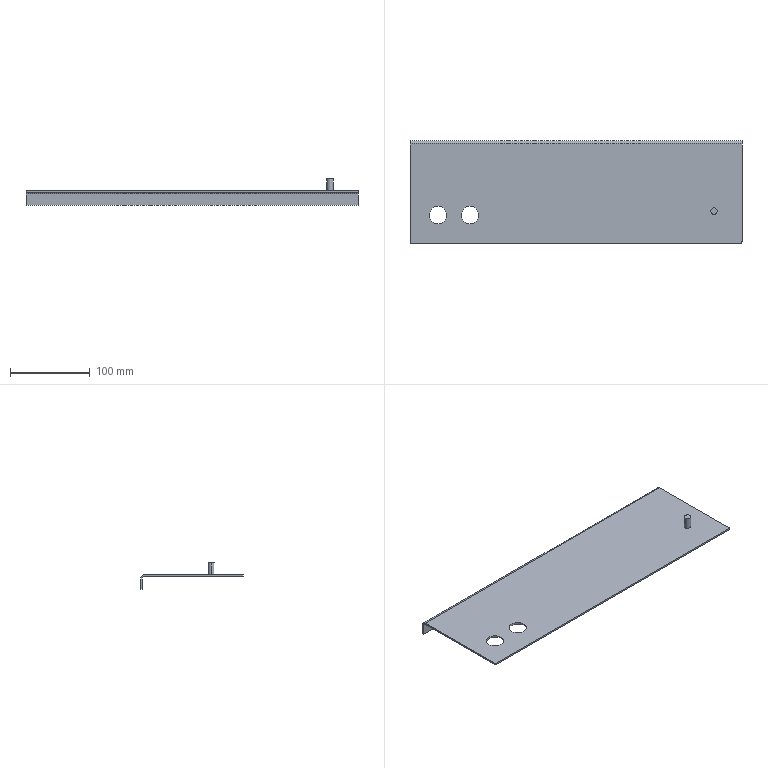Component | SolidWorks | ElectricalCabinetAssembly-1_CabinetAssembly-1_ElectricalCabinetBaffle-1 | 1 solid | 23 faces | box 415 x 128 x 33 mm | volume 117681 mm3 | plane 13 | cylinder 10 | commonest cylinder face diameters 22 x4 8 x3 4 x3 | material Plain Carbon Steel
STEP:
#1=COLOUR_RGB('',0.7922,0.8196,0.9333);
#2=FILL_AREA_STYLE_COLOUR('',#1);
#3=FILL_AREA_STYLE('',(#2));
#4=SURFACE_STYLE_FILL_AREA(#3);
#5=SURFACE_SIDE_STYLE('',(#4));
#6=SURFACE_STYLE_USAGE(.BOTH.,#5);
#7=PRESENTATION_STYLE_ASSIGNMENT((#6));
#8=CARTESIAN_POINT('',(94.303,43.919,55.885));
#9=VERTEX_POINT('',#8);
#10=CARTESIAN_POINT('',(93.988,43.919,55.885));
#11=VERTEX_POINT('',#10);
#12=CARTESIAN_POINT('',(94.145,43.919,55.885));
#13=DIRECTION('',(0.,-0.,1.));
#14=DIRECTION('',(1.,0.,0.));
#15=AXIS2_PLACEMENT_3D('',#12,#13,#14);
#16=CIRCLE('',#15,0.1575);
#17=EDGE_CURVE('',#9,#11,#16,.T.);
#18=ORIENTED_EDGE('',*,*,#17,.F.);
#19=CARTESIAN_POINT('',(94.303,43.919,55.294));
#20=VERTEX_POINT('',#19);
#21=CARTESIAN_POINT('',(94.303,43.919,55.885));
#22=DIRECTION('',(-0.,0.,-1.));
#23=VECTOR('',#22,39.37);
#24=LINE('',#21,#23);
#25=EDGE_CURVE('',#9,#20,#24,.T.);
#26=ORIENTED_EDGE('',*,*,#25,.T.);
#27=CARTESIAN_POINT('',(93.988,43.919,55.294));
#28=VERTEX_POINT('',#27);
#29=CARTESIAN_POINT('',(94.145,43.919,55.294));
#30=DIRECTION('',(0.,-0.,1.));
#31=DIRECTION('',(1.,0.,0.));
#32=AXIS2_PLACEMENT_3D('',#29,#30,#31);
#33=CIRCLE('',#32,0.1575);
#34=EDGE_CURVE('',#20,#28,#33,.T.);
#35=ORIENTED_EDGE('',*,*,#34,.T.);
#36=CARTESIAN_POINT('',(93.988,43.919,55.885));
#37=DIRECTION('',(-0.,0.,-1.));
#38=VECTOR('',#37,39.37);
#39=LINE('',#36,#38);
#40=EDGE_CURVE('',#11,#28,#39,.T.);
#41=ORIENTED_EDGE('',*,*,#40,.F.);
#42=EDGE_LOOP('',(#18,#26,#35,#41));
#43=FACE_OUTER_BOUND('',#42,.T.);
#44=CARTESIAN_POINT('',(94.145,43.919,55.885));
#45=DIRECTION('',(-0.,0.,-1.));
#46=DIRECTION('',(-1.,0.,0.));
#47=AXIS2_PLACEMENT_3D('',#44,#45,#46);
#48=CYLINDRICAL_SURFACE('',#47,0.1575);
#49=ADVANCED_FACE('',(#43),#48,.T.);
#50=CARTESIAN_POINT('',(81.704,43.722,55.216));
#51=VERTEX_POINT('',#50);
#52=CARTESIAN_POINT('',(82.57,43.722,55.216));
#53=VERTEX_POINT('',#52);
#54=CARTESIAN_POINT('',(82.137,43.722,55.216));
#55=DIRECTION('',(0.,-0.,1.));
#56=DIRECTION('',(1.,0.,0.));
#57=AXIS2_PLACEMENT_3D('',#54,#55,#56);
#58=CIRCLE('',#57,0.4331);
#59=EDGE_CURVE('',#51,#53,#58,.T.);
#60=ORIENTED_EDGE('',*,*,#59,.F.);
#61=CARTESIAN_POINT('',(81.704,43.722,55.294));
#62=VERTEX_POINT('',#61);
#63=CARTESIAN_POINT('',(81.704,43.722,54.901));
#64=DIRECTION('',(0.,-0.,1.));
#65=VECTOR('',#64,39.37);
#66=LINE('',#63,#65);
#67=EDGE_CURVE('',#51,#62,#66,.T.);
#68=ORIENTED_EDGE('',*,*,#67,.T.);
#69=CARTESIAN_POINT('',(82.57,43.722,55.294));
#70=VERTEX_POINT('',#69);
#71=CARTESIAN_POINT('',(82.137,43.722,55.294));
#72=DIRECTION('',(0.,-0.,1.));
#73=DIRECTION('',(1.,0.,0.));
#74=AXIS2_PLACEMENT_3D('',#71,#72,#73);
#75=CIRCLE('',#74,0.4331);
#76=EDGE_CURVE('',#62,#70,#75,.T.);
#77=ORIENTED_EDGE('',*,*,#76,.T.);
#78=CARTESIAN_POINT('',(82.57,43.722,54.901));
#79=DIRECTION('',(0.,-0.,1.));
#80=VECTOR('',#79,39.37);
#81=LINE('',#78,#80);
#82=EDGE_CURVE('',#53,#70,#81,.T.);
#83=ORIENTED_EDGE('',*,*,#82,.F.);
#84=EDGE_LOOP('',(#60,#68,#77,#83));
#85=FACE_OUTER_BOUND('',#84,.T.);
#86=CARTESIAN_POINT('',(82.137,43.722,54.901));
#87=DIRECTION('',(0.,-0.,1.));
#88=DIRECTION('',(1.,0.,0.));
#89=AXIS2_PLACEMENT_3D('',#86,#87,#88);
#90=CYLINDRICAL_SURFACE('',#89,0.4331);
#91=ADVANCED_FACE('',(#85),#90,.F.);
#92=CARTESIAN_POINT('',(80.129,43.722,55.216));
#93=VERTEX_POINT('',#92);
#94=CARTESIAN_POINT('',(80.996,43.722,55.216));
#95=VERTEX_POINT('',#94);
#96=CARTESIAN_POINT('',(80.562,43.722,55.216));
#97=DIRECTION('',(0.,-0.,1.));
#98=DIRECTION('',(1.,0.,0.));
#99=AXIS2_PLACEMENT_3D('',#96,#97,#98);
#100=CIRCLE('',#99,0.4331);
#101=EDGE_CURVE('',#93,#95,#100,.T.);
#102=ORIENTED_EDGE('',*,*,#101,.F.);
#103=CARTESIAN_POINT('',(80.129,43.722,55.294));
#104=VERTEX_POINT('',#103);
#105=CARTESIAN_POINT('',(80.129,43.722,54.901));
#106=DIRECTION('',(0.,-0.,1.));
#107=VECTOR('',#106,39.37);
#108=LINE('',#105,#107);
#109=EDGE_CURVE('',#93,#104,#108,.T.);
#110=ORIENTED_EDGE('',*,*,#109,.T.);
#111=CARTESIAN_POINT('',(80.996,43.722,55.294));
#112=VERTEX_POINT('',#111);
#113=CARTESIAN_POINT('',(80.562,43.722,55.294));
#114=DIRECTION('',(0.,-0.,1.));
#115=DIRECTION('',(1.,0.,0.));
#116=AXIS2_PLACEMENT_3D('',#113,#114,#115);
#117=CIRCLE('',#116,0.4331);
#118=EDGE_CURVE('',#104,#112,#117,.T.);
#119=ORIENTED_EDGE('',*,*,#118,.T.);
#120=CARTESIAN_POINT('',(80.996,43.722,54.901));
#121=DIRECTION('',(0.,-0.,1.));
#122=VECTOR('',#121,39.37);
#123=LINE('',#120,#122);
#124=EDGE_CURVE('',#95,#112,#123,.T.);
#125=ORIENTED_EDGE('',*,*,#124,.F.);
#126=EDGE_LOOP('',(#102,#110,#119,#125));
#127=FACE_OUTER_BOUND('',#126,.T.);
#128=CARTESIAN_POINT('',(80.562,43.722,54.901));
#129=DIRECTION('',(0.,-0.,1.));
#130=DIRECTION('',(1.,0.,0.));
#131=AXIS2_PLACEMENT_3D('',#128,#129,#130);
#132=CYLINDRICAL_SURFACE('',#131,0.4331);
#133=ADVANCED_FACE('',(#127),#132,.F.);
#134=CARTESIAN_POINT('',(95.523,47.226,55.216));
#135=VERTEX_POINT('',#134);
#136=CARTESIAN_POINT('',(95.523,42.423,55.216));
#137=VERTEX_POINT('',#136);
#138=CARTESIAN_POINT('',(95.523,42.423,55.216));
#139=DIRECTION('',(0.,-1.,-0.));
#140=VECTOR('',#139,39.37);
#141=LINE('',#138,#140);
#142=EDGE_CURVE('',#135,#137,#141,.T.);
#143=ORIENTED_EDGE('',*,*,#142,.F.);
#144=CARTESIAN_POINT('',(95.523,47.226,55.294));
#145=VERTEX_POINT('',#144);
#146=CARTESIAN_POINT('',(95.523,47.226,55.216));
#147=DIRECTION('',(0.,-0.,1.));
#148=VECTOR('',#147,39.37);
#149=LINE('',#146,#148);
#150=EDGE_CURVE('',#135,#145,#149,.T.);
#151=ORIENTED_EDGE('',*,*,#150,.T.);
#152=CARTESIAN_POINT('',(95.523,42.423,55.294));
#153=VERTEX_POINT('',#152);
#154=CARTESIAN_POINT('',(95.523,42.423,55.294));
#155=DIRECTION('',(0.,-1.,-0.));
#156=VECTOR('',#155,39.37);
#157=LINE('',#154,#156);
#158=EDGE_CURVE('',#145,#153,#157,.T.);
#159=ORIENTED_EDGE('',*,*,#158,.T.);
#160=CARTESIAN_POINT('',(95.523,42.423,55.294));
#161=DIRECTION('',(-0.,0.,-1.));
#162=VECTOR('',#161,39.37);
#163=LINE('',#160,#162);
#164=EDGE_CURVE('',#153,#137,#163,.T.);
#165=ORIENTED_EDGE('',*,*,#164,.T.);
#166=EDGE_LOOP('',(#143,#151,#159,#165));
#167=FACE_OUTER_BOUND('',#166,.T.);
#168=CARTESIAN_POINT('',(95.523,42.423,55.294));
#169=DIRECTION('',(1.,0.,-0.));
#170=DIRECTION('',(-0.,0.,-1.));
#171=AXIS2_PLACEMENT_3D('',#168,#169,#170);
#172=PLANE('',#171);
#173=ADVANCED_FACE('',(#167),#172,.T.);
#174=CARTESIAN_POINT('',(94.145,43.919,55.294));
#175=DIRECTION('',(0.,-0.,1.));
#176=DIRECTION('',(1.,0.,0.));
#177=AXIS2_PLACEMENT_3D('',#174,#175,#176);
#178=CIRCLE('',#177,0.1575);
#179=EDGE_CURVE('',#28,#20,#178,.T.);
#180=ORIENTED_EDGE('',*,*,#179,.F.);
#181=ORIENTED_EDGE('',*,*,#34,.F.);
#182=EDGE_LOOP('',(#180,#181));
#183=FACE_BOUND('',#182,.T.);
#184=CARTESIAN_POINT('',(82.137,43.722,55.294));
#185=DIRECTION('',(0.,-0.,1.));
#186=DIRECTION('',(1.,0.,0.));
#187=AXIS2_PLACEMENT_3D('',#184,#185,#186);
#188=CIRCLE('',#187,0.4331);
#189=EDGE_CURVE('',#70,#62,#188,.T.);
#190=ORIENTED_EDGE('',*,*,#189,.F.);
#191=ORIENTED_EDGE('',*,*,#76,.F.);
#192=EDGE_LOOP('',(#190,#191));
#193=FACE_BOUND('',#192,.T.);
#194=CARTESIAN_POINT('',(80.562,43.722,55.294));
#195=DIRECTION('',(0.,-0.,1.));
#196=DIRECTION('',(1.,0.,0.));
#197=AXIS2_PLACEMENT_3D('',#194,#195,#196);
#198=CIRCLE('',#197,0.4331);
#199=EDGE_CURVE('',#112,#104,#198,.T.);
#200=ORIENTED_EDGE('',*,*,#199,.F.);
#201=ORIENTED_EDGE('',*,*,#118,.F.);
#202=EDGE_LOOP('',(#200,#201));
#203=FACE_BOUND('',#202,.T.);
#204=ORIENTED_EDGE('',*,*,#158,.F.);
#205=CARTESIAN_POINT('',(79.185,47.226,55.294));
#206=VERTEX_POINT('',#205);
#207=CARTESIAN_POINT('',(95.523,47.226,55.294));
#208=DIRECTION('',(-1.,-0.,0.));
#209=VECTOR('',#208,39.37);
#210=LINE('',#207,#209);
#211=EDGE_CURVE('',#145,#206,#210,.T.);
#212=ORIENTED_EDGE('',*,*,#211,.T.);
#213=CARTESIAN_POINT('',(79.185,42.423,55.294));
#214=VERTEX_POINT('',#213);
#215=CARTESIAN_POINT('',(79.185,42.423,55.294));
#216=DIRECTION('',(-0.,1.,0.));
#217=VECTOR('',#216,39.37);
#218=LINE('',#215,#217);
#219=EDGE_CURVE('',#214,#206,#218,.T.);
#220=ORIENTED_EDGE('',*,*,#219,.F.);
#221=CARTESIAN_POINT('',(79.263,42.344,55.294));
#222=VERTEX_POINT('',#221);
#223=CARTESIAN_POINT('',(79.263,42.423,55.294));
#224=DIRECTION('',(-0.,0.,-1.));
#225=DIRECTION('',(1.,0.,0.));
#226=AXIS2_PLACEMENT_3D('',#223,#224,#225);
#227=CIRCLE('',#226,0.07874);
#228=EDGE_CURVE('',#222,#214,#227,.T.);
#229=ORIENTED_EDGE('',*,*,#228,.F.);
#230=CARTESIAN_POINT('',(95.444,42.344,55.294));
#231=VERTEX_POINT('',#230);
#232=CARTESIAN_POINT('',(95.444,42.344,55.294));
#233=DIRECTION('',(-1.,-0.,0.));
#234=VECTOR('',#233,39.37);
#235=LINE('',#232,#234);
#236=EDGE_CURVE('',#231,#222,#235,.T.);
#237=ORIENTED_EDGE('',*,*,#236,.F.);
#238=CARTESIAN_POINT('',(95.444,42.423,55.294));
#239=DIRECTION('',(-0.,0.,-1.));
#240=DIRECTION('',(1.,0.,0.));
#241=AXIS2_PLACEMENT_3D('',#238,#239,#240);
#242=CIRCLE('',#241,0.07874);
#243=EDGE_CURVE('',#153,#231,#242,.T.);
#244=ORIENTED_EDGE('',*,*,#243,.F.);
#245=EDGE_LOOP('',(#204,#212,#220,#229,#237,#244));
#246=FACE_OUTER_BOUND('',#245,.T.);
#247=CARTESIAN_POINT('',(95.444,42.423,55.294));
#248=DIRECTION('',(0.,-0.,1.));
#249=DIRECTION('',(1.,0.,-0.));
#250=AXIS2_PLACEMENT_3D('',#247,#248,#249);
#251=PLANE('',#250);
#252=ADVANCED_FACE('',(#183,#193,#203,#246),#251,.T.);
#253=CARTESIAN_POINT('',(82.137,43.722,55.216));
#254=DIRECTION('',(0.,-0.,1.));
#255=DIRECTION('',(1.,0.,0.));
#256=AXIS2_PLACEMENT_3D('',#253,#254,#255);
#257=CIRCLE('',#256,0.4331);
#258=EDGE_CURVE('',#53,#51,#257,.T.);
#259=ORIENTED_EDGE('',*,*,#258,.T.);
#260=ORIENTED_EDGE('',*,*,#59,.T.);
#261=EDGE_LOOP('',(#259,#260));
#262=FACE_BOUND('',#261,.T.);
#263=CARTESIAN_POINT('',(80.562,43.722,55.216));
#264=DIRECTION('',(0.,-0.,1.));
#265=DIRECTION('',(1.,0.,0.));
#266=AXIS2_PLACEMENT_3D('',#263,#264,#265);
#267=CIRCLE('',#266,0.4331);
#268=EDGE_CURVE('',#95,#93,#267,.T.);
#269=ORIENTED_EDGE('',*,*,#268,.T.);
#270=ORIENTED_EDGE('',*,*,#101,.T.);
#271=EDGE_LOOP('',(#269,#270));
#272=FACE_BOUND('',#271,.T.);
#273=CARTESIAN_POINT('',(79.185,47.226,55.216));
#274=VERTEX_POINT('',#273);
#275=CARTESIAN_POINT('',(95.523,47.226,55.216));
#276=DIRECTION('',(-1.,-0.,0.));
#277=VECTOR('',#276,39.37);
#278=LINE('',#275,#277);
#279=EDGE_CURVE('',#135,#274,#278,.T.);
#280=ORIENTED_EDGE('',*,*,#279,.F.);
#281=ORIENTED_EDGE('',*,*,#142,.T.);
#282=CARTESIAN_POINT('',(95.444,42.344,55.216));
#283=VERTEX_POINT('',#282);
#284=CARTESIAN_POINT('',(95.444,42.423,55.216));
#285=DIRECTION('',(-0.,0.,-1.));
#286=DIRECTION('',(1.,0.,0.));
#287=AXIS2_PLACEMENT_3D('',#284,#285,#286);
#288=CIRCLE('',#287,0.07874);
#289=EDGE_CURVE('',#137,#283,#288,.T.);
#290=ORIENTED_EDGE('',*,*,#289,.T.);
#291=CARTESIAN_POINT('',(79.263,42.344,55.216));
#292=VERTEX_POINT('',#291);
#293=CARTESIAN_POINT('',(95.444,42.344,55.216));
#294=DIRECTION('',(-1.,-0.,0.));
#295=VECTOR('',#294,39.37);
#296=LINE('',#293,#295);
#297=EDGE_CURVE('',#283,#292,#296,.T.);
#298=ORIENTED_EDGE('',*,*,#297,.T.);
#299=CARTESIAN_POINT('',(79.185,42.423,55.216));
#300=VERTEX_POINT('',#299);
#301=CARTESIAN_POINT('',(79.263,42.423,55.216));
#302=DIRECTION('',(-0.,0.,-1.));
#303=DIRECTION('',(1.,0.,0.));
#304=AXIS2_PLACEMENT_3D('',#301,#302,#303);
#305=CIRCLE('',#304,0.07874);
#306=EDGE_CURVE('',#292,#300,#305,.T.);
#307=ORIENTED_EDGE('',*,*,#306,.T.);
#308=CARTESIAN_POINT('',(79.185,42.423,55.216));
#309=DIRECTION('',(-0.,1.,0.));
#310=VECTOR('',#309,39.37);
#311=LINE('',#308,#310);
#312=EDGE_CURVE('',#300,#274,#311,.T.);
#313=ORIENTED_EDGE('',*,*,#312,.T.);
#314=EDGE_LOOP('',(#280,#281,#290,#298,#307,#313));
#315=FACE_OUTER_BOUND('',#314,.T.);
#316=CARTESIAN_POINT('',(95.444,42.423,55.216));
#317=DIRECTION('',(0.,-0.,1.));
#318=DIRECTION('',(1.,0.,-0.));
#319=AXIS2_PLACEMENT_3D('',#316,#317,#318);
#320=PLANE('',#319);
#321=ADVANCED_FACE('',(#262,#272,#315),#320,.F.);
#322=CARTESIAN_POINT('',(79.185,47.226,55.216));
#323=DIRECTION('',(0.,-0.,1.));
#324=VECTOR('',#323,39.37);
#325=LINE('',#322,#324);
#326=EDGE_CURVE('',#274,#206,#325,.T.);
#327=ORIENTED_EDGE('',*,*,#326,.F.);
#328=ORIENTED_EDGE('',*,*,#312,.F.);
#329=CARTESIAN_POINT('',(79.185,42.423,55.294));
#330=DIRECTION('',(-0.,0.,-1.));
#331=VECTOR('',#330,39.37);
#332=LINE('',#329,#331);
#333=EDGE_CURVE('',#214,#300,#332,.T.);
#334=ORIENTED_EDGE('',*,*,#333,.F.);
#335=ORIENTED_EDGE('',*,*,#219,.T.);
#336=EDGE_LOOP('',(#327,#328,#334,#335));
#337=FACE_OUTER_BOUND('',#336,.T.);
#338=CARTESIAN_POINT('',(79.185,42.423,55.294));
#339=DIRECTION('',(-1.,-0.,0.));
#340=DIRECTION('',(0.,-0.,1.));
#341=AXIS2_PLACEMENT_3D('',#338,#339,#340);
#342=PLANE('',#341);
#343=ADVANCED_FACE('',(#337),#342,.T.);
#344=ORIENTED_EDGE('',*,*,#306,.F.);
#345=CARTESIAN_POINT('',(79.263,42.344,55.294));
#346=DIRECTION('',(-0.,0.,-1.));
#347=VECTOR('',#346,39.37);
#348=LINE('',#345,#347);
#349=EDGE_CURVE('',#222,#292,#348,.T.);
#350=ORIENTED_EDGE('',*,*,#349,.F.);
#351=ORIENTED_EDGE('',*,*,#228,.T.);
#352=ORIENTED_EDGE('',*,*,#333,.T.);
#353=EDGE_LOOP('',(#344,#350,#351,#352));
#354=FACE_OUTER_BOUND('',#353,.T.);
#355=CARTESIAN_POINT('',(79.263,42.423,55.294));
#356=DIRECTION('',(-0.,0.,-1.));
#357=DIRECTION('',(-1.,0.,0.));
#358=AXIS2_PLACEMENT_3D('',#355,#356,#357);
#359=CYLINDRICAL_SURFACE('',#358,0.07874);
#360=ADVANCED_FACE('',(#354),#359,.T.);
#361=ORIENTED_EDGE('',*,*,#297,.F.);
#362=CARTESIAN_POINT('',(95.444,42.344,55.294));
#363=DIRECTION('',(-0.,0.,-1.));
#364=VECTOR('',#363,39.37);
#365=LINE('',#362,#364);
#366=EDGE_CURVE('',#231,#283,#365,.T.);
#367=ORIENTED_EDGE('',*,*,#366,.F.);
#368=ORIENTED_EDGE('',*,*,#236,.T.);
#369=ORIENTED_EDGE('',*,*,#349,.T.);
#370=EDGE_LOOP('',(#361,#367,#368,#369));
#371=FACE_OUTER_BOUND('',#370,.T.);
#372=CARTESIAN_POINT('',(95.444,42.344,55.294));
#373=DIRECTION('',(0.,-1.,-0.));
#374=DIRECTION('',(0.,-0.,1.));
#375=AXIS2_PLACEMENT_3D('',#372,#373,#374);
#376=PLANE('',#375);
#377=ADVANCED_FACE('',(#371),#376,.T.);
#378=ORIENTED_EDGE('',*,*,#289,.F.);
#379=ORIENTED_EDGE('',*,*,#164,.F.);
#380=ORIENTED_EDGE('',*,*,#243,.T.);
#381=ORIENTED_EDGE('',*,*,#366,.T.);
#382=EDGE_LOOP('',(#378,#379,#380,#381));
#383=FACE_OUTER_BOUND('',#382,.T.);
#384=CARTESIAN_POINT('',(95.444,42.423,55.294));
#385=DIRECTION('',(-0.,0.,-1.));
#386=DIRECTION('',(-1.,0.,0.));
#387=AXIS2_PLACEMENT_3D('',#384,#385,#386);
#388=CYLINDRICAL_SURFACE('',#387,0.07874);
#389=ADVANCED_FACE('',(#383),#388,.T.);
#390=CARTESIAN_POINT('',(79.185,47.305,55.137));
#391=VERTEX_POINT('',#390);
#392=CARTESIAN_POINT('',(79.185,47.384,55.137));
#393=VERTEX_POINT('',#392);
#394=CARTESIAN_POINT('',(79.185,47.384,55.137));
#395=DIRECTION('',(-0.,1.,0.));
#396=VECTOR('',#395,39.37);
#397=LINE('',#394,#396);
#398=EDGE_CURVE('',#391,#393,#397,.T.);
#399=ORIENTED_EDGE('',*,*,#398,.F.);
#400=CARTESIAN_POINT('',(79.185,47.226,55.137));
#401=DIRECTION('',(-1.,-0.,0.));
#402=DIRECTION('',(0.,0.,-1.));
#403=AXIS2_PLACEMENT_3D('',#400,#401,#402);
#404=CIRCLE('',#403,0.07874);
#405=EDGE_CURVE('',#274,#391,#404,.T.);
#406=ORIENTED_EDGE('',*,*,#405,.F.);
#407=ORIENTED_EDGE('',*,*,#326,.T.);
#408=CARTESIAN_POINT('',(79.185,47.226,55.137));
#409=DIRECTION('',(-1.,-0.,0.));
#410=DIRECTION('',(0.,0.,-1.));
#411=AXIS2_PLACEMENT_3D('',#408,#409,#410);
#412=CIRCLE('',#411,0.1575);
#413=EDGE_CURVE('',#206,#393,#412,.T.);
#414=ORIENTED_EDGE('',*,*,#413,.T.);
#415=EDGE_LOOP('',(#399,#406,#407,#414));
#416=FACE_OUTER_BOUND('',#415,.T.);
#417=CARTESIAN_POINT('',(79.185,47.226,55.137));
#418=DIRECTION('',(-1.,-0.,0.));
#419=DIRECTION('',(0.,-0.,1.));
#420=AXIS2_PLACEMENT_3D('',#417,#418,#419);
#421=PLANE('',#420);
#422=ADVANCED_FACE('',(#416),#421,.T.);
#423=CARTESIAN_POINT('',(95.523,47.305,55.137));
#424=VERTEX_POINT('',#423);
#425=CARTESIAN_POINT('',(95.523,47.226,55.137));
#426=DIRECTION('',(1.,0.,-0.));
#427=DIRECTION('',(0.,0.,-1.));
#428=AXIS2_PLACEMENT_3D('',#425,#426,#427);
#429=CIRCLE('',#428,0.07874);
#430=EDGE_CURVE('',#424,#135,#429,.T.);
#431=ORIENTED_EDGE('',*,*,#430,.F.);
#432=CARTESIAN_POINT('',(95.523,47.384,55.137));
#433=VERTEX_POINT('',#432);
#434=CARTESIAN_POINT('',(95.523,47.305,55.137));
#435=DIRECTION('',(-0.,1.,0.));
#436=VECTOR('',#435,39.37);
#437=LINE('',#434,#436);
#438=EDGE_CURVE('',#424,#433,#437,.T.);
#439=ORIENTED_EDGE('',*,*,#438,.T.);
#440=CARTESIAN_POINT('',(95.523,47.226,55.137));
#441=DIRECTION('',(1.,0.,-0.));
#442=DIRECTION('',(0.,0.,-1.));
#443=AXIS2_PLACEMENT_3D('',#440,#441,#442);
#444=CIRCLE('',#443,0.1575);
#445=EDGE_CURVE('',#433,#145,#444,.T.);
#446=ORIENTED_EDGE('',*,*,#445,.T.);
#447=ORIENTED_EDGE('',*,*,#150,.F.);
#448=EDGE_LOOP('',(#431,#439,#446,#447));
#449=FACE_OUTER_BOUND('',#448,.T.);
#450=CARTESIAN_POINT('',(95.523,47.226,55.137));
#451=DIRECTION('',(-1.,-0.,0.));
#452=DIRECTION('',(0.,-0.,1.));
#453=AXIS2_PLACEMENT_3D('',#450,#451,#452);
#454=PLANE('',#453);
#455=ADVANCED_FACE('',(#449),#454,.F.);
#456=ORIENTED_EDGE('',*,*,#211,.F.);
#457=ORIENTED_EDGE('',*,*,#445,.F.);
#458=CARTESIAN_POINT('',(79.185,47.384,55.137));
#459=DIRECTION('',(-1.,-0.,0.));
#460=VECTOR('',#459,39.37);
#461=LINE('',#458,#460);
#462=EDGE_CURVE('',#433,#393,#461,.T.);
#463=ORIENTED_EDGE('',*,*,#462,.T.);
#464=ORIENTED_EDGE('',*,*,#413,.F.);
#465=EDGE_LOOP('',(#456,#457,#463,#464));
#466=FACE_OUTER_BOUND('',#465,.T.);
#467=CARTESIAN_POINT('',(95.523,47.226,55.137));
#468=DIRECTION('',(1.,0.,-0.));
#469=DIRECTION('',(0.,1.,0.));
#470=AXIS2_PLACEMENT_3D('',#467,#468,#469);
#471=CYLINDRICAL_SURFACE('',#470,0.1575);
#472=ADVANCED_FACE('',(#466),#471,.T.);
#473=ORIENTED_EDGE('',*,*,#279,.T.);
#474=ORIENTED_EDGE('',*,*,#405,.T.);
#475=CARTESIAN_POINT('',(79.185,47.305,55.137));
#476=DIRECTION('',(1.,0.,-0.));
#477=VECTOR('',#476,39.37);
#478=LINE('',#475,#477);
#479=EDGE_CURVE('',#391,#424,#478,.T.);
#480=ORIENTED_EDGE('',*,*,#479,.T.);
#481=ORIENTED_EDGE('',*,*,#430,.T.);
#482=EDGE_LOOP('',(#473,#474,#480,#481));
#483=FACE_OUTER_BOUND('',#482,.T.);
#484=CARTESIAN_POINT('',(95.523,47.226,55.137));
#485=DIRECTION('',(1.,0.,-0.));
#486=DIRECTION('',(0.,1.,0.));
#487=AXIS2_PLACEMENT_3D('',#484,#485,#486);
#488=CYLINDRICAL_SURFACE('',#487,0.07874);
#489=ADVANCED_FACE('',(#483),#488,.F.);
#490=ORIENTED_EDGE('',*,*,#438,.F.);
#491=CARTESIAN_POINT('',(95.523,47.305,54.586));
#492=VERTEX_POINT('',#491);
#493=CARTESIAN_POINT('',(95.523,47.305,54.586));
#494=DIRECTION('',(-0.,0.,-1.));
#495=VECTOR('',#494,39.37);
#496=LINE('',#493,#495);
#497=EDGE_CURVE('',#424,#492,#496,.T.);
#498=ORIENTED_EDGE('',*,*,#497,.T.);
#499=CARTESIAN_POINT('',(95.523,47.384,54.586));
#500=VERTEX_POINT('',#499);
#501=CARTESIAN_POINT('',(95.523,47.384,54.586));
#502=DIRECTION('',(0.,-1.,-0.));
#503=VECTOR('',#502,39.37);
#504=LINE('',#501,#503);
#505=EDGE_CURVE('',#500,#492,#504,.T.);
#506=ORIENTED_EDGE('',*,*,#505,.F.);
#507=CARTESIAN_POINT('',(95.523,47.384,55.216));
#508=DIRECTION('',(-0.,0.,-1.));
#509=VECTOR('',#508,39.37);
#510=LINE('',#507,#509);
#511=EDGE_CURVE('',#433,#500,#510,.T.);
#512=ORIENTED_EDGE('',*,*,#511,.F.);
#513=EDGE_LOOP('',(#490,#498,#506,#512));
#514=FACE_OUTER_BOUND('',#513,.T.);
#515=CARTESIAN_POINT('',(95.523,47.384,54.586));
#516=DIRECTION('',(-1.,-0.,0.));
#517=DIRECTION('',(0.,-0.,1.));
#518=AXIS2_PLACEMENT_3D('',#515,#516,#517);
#519=PLANE('',#518);
#520=ADVANCED_FACE('',(#514),#519,.F.);
#521=ORIENTED_EDGE('',*,*,#398,.T.);
#522=CARTESIAN_POINT('',(79.185,47.384,54.586));
#523=VERTEX_POINT('',#522);
#524=CARTESIAN_POINT('',(79.185,47.384,55.216));
#525=DIRECTION('',(0.,-0.,1.));
#526=VECTOR('',#525,39.37);
#527=LINE('',#524,#526);
#528=EDGE_CURVE('',#523,#393,#527,.T.);
#529=ORIENTED_EDGE('',*,*,#528,.F.);
#530=CARTESIAN_POINT('',(79.185,47.305,54.586));
#531=VERTEX_POINT('',#530);
#532=CARTESIAN_POINT('',(79.185,47.384,54.586));
#533=DIRECTION('',(0.,-1.,-0.));
#534=VECTOR('',#533,39.37);
#535=LINE('',#532,#534);
#536=EDGE_CURVE('',#523,#531,#535,.T.);
#537=ORIENTED_EDGE('',*,*,#536,.T.);
#538=CARTESIAN_POINT('',(79.185,47.305,55.216));
#539=DIRECTION('',(0.,-0.,1.));
#540=VECTOR('',#539,39.37);
#541=LINE('',#538,#540);
#542=EDGE_CURVE('',#531,#391,#541,.T.);
#543=ORIENTED_EDGE('',*,*,#542,.T.);
#544=EDGE_LOOP('',(#521,#529,#537,#543));
#545=FACE_OUTER_BOUND('',#544,.T.);
#546=CARTESIAN_POINT('',(79.185,47.384,55.216));
#547=DIRECTION('',(1.,0.,-0.));
#548=DIRECTION('',(-0.,0.,-1.));
#549=AXIS2_PLACEMENT_3D('',#546,#547,#548);
#550=PLANE('',#549);
#551=ADVANCED_FACE('',(#545),#550,.F.);
#552=ORIENTED_EDGE('',*,*,#462,.F.);
#553=ORIENTED_EDGE('',*,*,#511,.T.);
#554=CARTESIAN_POINT('',(95.523,47.384,54.586));
#555=DIRECTION('',(-1.,-0.,0.));
#556=VECTOR('',#555,39.37);
#557=LINE('',#554,#556);
#558=EDGE_CURVE('',#500,#523,#557,.T.);
#559=ORIENTED_EDGE('',*,*,#558,.T.);
#560=ORIENTED_EDGE('',*,*,#528,.T.);
#561=EDGE_LOOP('',(#552,#553,#559,#560));
#562=FACE_OUTER_BOUND('',#561,.T.);
#563=CARTESIAN_POINT('',(95.523,47.384,55.216));
#564=DIRECTION('',(0.,-1.,-0.));
#565=DIRECTION('',(0.,-0.,1.));
#566=AXIS2_PLACEMENT_3D('',#563,#564,#565);
#567=PLANE('',#566);
#568=ADVANCED_FACE('',(#562),#567,.F.);
#569=ORIENTED_EDGE('',*,*,#497,.F.);
#570=ORIENTED_EDGE('',*,*,#479,.F.);
#571=ORIENTED_EDGE('',*,*,#542,.F.);
#572=CARTESIAN_POINT('',(79.185,47.305,54.586));
#573=DIRECTION('',(-1.,-0.,0.));
#574=VECTOR('',#573,39.37);
#575=LINE('',#572,#574);
#576=EDGE_CURVE('',#492,#531,#575,.T.);
#577=ORIENTED_EDGE('',*,*,#576,.F.);
#578=EDGE_LOOP('',(#569,#570,#571,#577));
#579=FACE_OUTER_BOUND('',#578,.T.);
#580=CARTESIAN_POINT('',(95.523,47.305,55.216));
#581=DIRECTION('',(0.,-1.,-0.));
#582=DIRECTION('',(0.,-0.,1.));
#583=AXIS2_PLACEMENT_3D('',#580,#581,#582);
#584=PLANE('',#583);
#585=ADVANCED_FACE('',(#579),#584,.T.);
#586=ORIENTED_EDGE('',*,*,#576,.T.);
#587=ORIENTED_EDGE('',*,*,#536,.F.);
#588=ORIENTED_EDGE('',*,*,#558,.F.);
#589=ORIENTED_EDGE('',*,*,#505,.T.);
#590=EDGE_LOOP('',(#586,#587,#588,#589));
#591=FACE_OUTER_BOUND('',#590,.T.);
#592=CARTESIAN_POINT('',(79.185,47.384,54.586));
#593=DIRECTION('',(0.,-0.,1.));
#594=DIRECTION('',(-0.,1.,0.));
#595=AXIS2_PLACEMENT_3D('',#592,#593,#594);
#596=PLANE('',#595);
#597=ADVANCED_FACE('',(#591),#596,.F.);
#598=ORIENTED_EDGE('',*,*,#109,.F.);
#599=ORIENTED_EDGE('',*,*,#268,.F.);
#600=ORIENTED_EDGE('',*,*,#124,.T.);
#601=ORIENTED_EDGE('',*,*,#199,.T.);
#602=EDGE_LOOP('',(#598,#599,#600,#601));
#603=FACE_OUTER_BOUND('',#602,.T.);
#604=CARTESIAN_POINT('',(80.562,43.722,54.901));
#605=DIRECTION('',(0.,-0.,1.));
#606=DIRECTION('',(1.,0.,0.));
#607=AXIS2_PLACEMENT_3D('',#604,#605,#606);
#608=CYLINDRICAL_SURFACE('',#607,0.4331);
#609=ADVANCED_FACE('',(#603),#608,.F.);
#610=ORIENTED_EDGE('',*,*,#67,.F.);
#611=ORIENTED_EDGE('',*,*,#258,.F.);
#612=ORIENTED_EDGE('',*,*,#82,.T.);
#613=ORIENTED_EDGE('',*,*,#189,.T.);
#614=EDGE_LOOP('',(#610,#611,#612,#613));
#615=FACE_OUTER_BOUND('',#614,.T.);
#616=CARTESIAN_POINT('',(82.137,43.722,54.901));
#617=DIRECTION('',(0.,-0.,1.));
#618=DIRECTION('',(1.,0.,0.));
#619=AXIS2_PLACEMENT_3D('',#616,#617,#618);
#620=CYLINDRICAL_SURFACE('',#619,0.4331);
#621=ADVANCED_FACE('',(#615),#620,.F.);
#622=ORIENTED_EDGE('',*,*,#25,.F.);
#623=CARTESIAN_POINT('',(94.145,43.919,55.885));
#624=DIRECTION('',(0.,-0.,1.));
#625=DIRECTION('',(1.,0.,0.));
#626=AXIS2_PLACEMENT_3D('',#623,#624,#625);
#627=CIRCLE('',#626,0.1575);
#628=EDGE_CURVE('',#11,#9,#627,.T.);
#629=ORIENTED_EDGE('',*,*,#628,.F.);
#630=ORIENTED_EDGE('',*,*,#40,.T.);
#631=ORIENTED_EDGE('',*,*,#179,.T.);
#632=EDGE_LOOP('',(#622,#629,#630,#631));
#633=FACE_OUTER_BOUND('',#632,.T.);
#634=CARTESIAN_POINT('',(94.145,43.919,55.885));
#635=DIRECTION('',(-0.,0.,-1.));
#636=DIRECTION('',(-1.,0.,0.));
#637=AXIS2_PLACEMENT_3D('',#634,#635,#636);
#638=CYLINDRICAL_SURFACE('',#637,0.1575);
#639=ADVANCED_FACE('',(#633),#638,.T.);
#640=ORIENTED_EDGE('',*,*,#628,.T.);
#641=ORIENTED_EDGE('',*,*,#17,.T.);
#642=EDGE_LOOP('',(#640,#641));
#643=FACE_OUTER_BOUND('',#642,.T.);
#644=CARTESIAN_POINT('',(94.145,43.919,55.885));
#645=DIRECTION('',(0.,-0.,1.));
#646=DIRECTION('',(1.,0.,-0.));
#647=AXIS2_PLACEMENT_3D('',#644,#645,#646);
#648=PLANE('',#647);
#649=ADVANCED_FACE('',(#643),#648,.T.);
#650=CLOSED_SHELL('',(#49,#91,#133,#173,#252,#321,#343,#360,#377,#389,#422,#455,#472,#489,#520,#551,#568,#585,#597,#609,#621,#639,#649));
#651=MANIFOLD_SOLID_BREP('',#650);
#652=STYLED_ITEM('',(#7),#651);
#653=(LENGTH_UNIT()NAMED_UNIT(*)SI_UNIT($,.METRE.));
#654=LENGTH_MEASURE_WITH_UNIT(LENGTH_MEASURE(0.0254),#653);
#655=DIMENSIONAL_EXPONENTS(1.,0.,0.,0.,0.,0.,0.);
#656=(CONVERSION_BASED_UNIT('',#654)LENGTH_UNIT()NAMED_UNIT(#655));
#657=UNCERTAINTY_MEASURE_WITH_UNIT(LENGTH_MEASURE(0.00001),#656,'','');
#658=(NAMED_UNIT(*)PLANE_ANGLE_UNIT()SI_UNIT($,.RADIAN.));
#659=(NAMED_UNIT(*)SI_UNIT($,.STERADIAN.)SOLID_ANGLE_UNIT());
#660=(GEOMETRIC_REPRESENTATION_CONTEXT(3)GLOBAL_UNCERTAINTY_ASSIGNED_CONTEXT((#657))GLOBAL_UNIT_ASSIGNED_CONTEXT((#656,#658,#659))REPRESENTATION_CONTEXT('',''));
#661=MECHANICAL_DESIGN_GEOMETRIC_PRESENTATION_REPRESENTATION('',(#652),#660);
#662=CARTESIAN_POINT('',(0.,0.,0.));
#663=DIRECTION('',(0.,0.,1.));
#664=DIRECTION('',(1.,0.,0.));
#665=AXIS2_PLACEMENT_3D('',#662,#663,#664);
#666=(LENGTH_UNIT()NAMED_UNIT(*)SI_UNIT($,.METRE.));
#667=LENGTH_MEASURE_WITH_UNIT(LENGTH_MEASURE(0.0254),#666);
#668=DIMENSIONAL_EXPONENTS(1.,0.,0.,0.,0.,0.,0.);
#669=(CONVERSION_BASED_UNIT('',#667)LENGTH_UNIT()NAMED_UNIT(#668));
#670=UNCERTAINTY_MEASURE_WITH_UNIT(LENGTH_MEASURE(0.00001),#669,'','');
#671=(NAMED_UNIT(*)PLANE_ANGLE_UNIT()SI_UNIT($,.RADIAN.));
#672=(NAMED_UNIT(*)SI_UNIT($,.STERADIAN.)SOLID_ANGLE_UNIT());
#673=(GEOMETRIC_REPRESENTATION_CONTEXT(3)GLOBAL_UNCERTAINTY_ASSIGNED_CONTEXT((#670))GLOBAL_UNIT_ASSIGNED_CONTEXT((#669,#671,#672))REPRESENTATION_CONTEXT('',''));
#674=ADVANCED_BREP_SHAPE_REPRESENTATION('',(#651,#665),#673);
#675=PRESENTATION_LAYER_ASSIGNMENT('','',(#652));